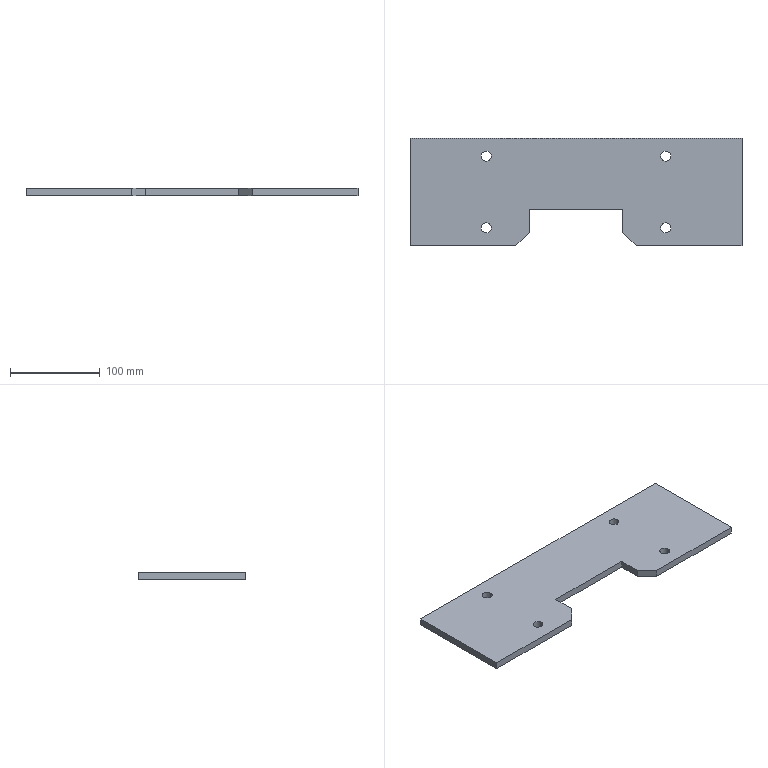Component | SolidWorks | THK-A1021FrontEndConnectingPlate-1 | 1 solid | 20 faces | box 370 x 120 x 8 mm | volume 317079 mm3 | plane 12 | cylinder 8 | commonest cylinder face diameters 11 x8 | material Q235A
build123d program:
from build123d import *

# Parameters (mm, degrees)
BOSS_EXTRUDE1_DEPTH        = 4
F_11_0_11_DIAMETER_HOLE1_D = 11
CHAMFER1_SIZE              = 15


with BuildPart() as part:
    # Sketch1 → Boss-Extrude1 (new, symmetric)
    with BuildSketch(Plane.XY):
        Polygon((-185, 60), (185, 60), (185, -60), (52, -60), (52, -20), (-52, -20), (-52, -60), (-185, -60), align=None)
    extrude(amount=BOSS_EXTRUDE1_DEPTH, both=True)

    # 11.0 _11_ Diameter Hole1 (through all)
    with Locations(Plane.XY.offset(4)):
        with Locations((-100, 40), (100, 40), (-100, -40), (100, -40)):
            Hole(F_11_0_11_DIAMETER_HOLE1_D / 2)

    # Chamfer1
    chamfer1_edges = [part.edges().sort_by_distance(p)[0] for p in [
        (52, -60, 0),
        (-52, -60, 0),
    ]]
    chamfer(chamfer1_edges, length=CHAMFER1_SIZE)


solid = part.part

# Placed as in the assembly
solid = solid.moved(Location((0, -115, -1245), (0, 0, 0)))
STEP:
#1=CARTESIAN_POINT('',(-4.154,-2.953,-49.173));
#2=VERTEX_POINT('',#1);
#3=CARTESIAN_POINT('',(-3.72,-2.953,-49.173));
#4=VERTEX_POINT('',#3);
#5=CARTESIAN_POINT('',(-3.937,-2.953,-49.173));
#6=DIRECTION('',(0.,0.,1.));
#7=DIRECTION('',(1.,0.,0.));
#8=AXIS2_PLACEMENT_3D('',#5,#6,#7);
#9=CIRCLE('',#8,0.2165);
#10=EDGE_CURVE('',#2,#4,#9,.T.);
#11=ORIENTED_EDGE('',*,*,#10,.F.);
#12=CARTESIAN_POINT('',(-4.154,-2.953,-48.858));
#13=VERTEX_POINT('',#12);
#14=CARTESIAN_POINT('',(-4.154,-2.953,-48.858));
#15=DIRECTION('',(0.,0.,1.));
#16=VECTOR('',#15,39.37);
#17=LINE('',#14,#16);
#18=EDGE_CURVE('',#2,#13,#17,.T.);
#19=ORIENTED_EDGE('',*,*,#18,.T.);
#20=CARTESIAN_POINT('',(-3.72,-2.953,-48.858));
#21=VERTEX_POINT('',#20);
#22=CARTESIAN_POINT('',(-3.937,-2.953,-48.858));
#23=DIRECTION('',(0.,0.,1.));
#24=DIRECTION('',(1.,0.,0.));
#25=AXIS2_PLACEMENT_3D('',#22,#23,#24);
#26=CIRCLE('',#25,0.2165);
#27=EDGE_CURVE('',#13,#21,#26,.T.);
#28=ORIENTED_EDGE('',*,*,#27,.T.);
#29=CARTESIAN_POINT('',(-3.72,-2.953,-48.858));
#30=DIRECTION('',(0.,0.,1.));
#31=VECTOR('',#30,39.37);
#32=LINE('',#29,#31);
#33=EDGE_CURVE('',#4,#21,#32,.T.);
#34=ORIENTED_EDGE('',*,*,#33,.F.);
#35=EDGE_LOOP('',(#11,#19,#28,#34));
#36=FACE_OUTER_BOUND('',#35,.T.);
#37=CARTESIAN_POINT('',(-3.937,-2.953,-48.858));
#38=DIRECTION('',(0.,0.,1.));
#39=DIRECTION('',(1.,0.,0.));
#40=AXIS2_PLACEMENT_3D('',#37,#38,#39);
#41=CYLINDRICAL_SURFACE('',#40,0.2165);
#42=ADVANCED_FACE('',(#36),#41,.F.);
#43=CARTESIAN_POINT('',(3.72,-2.953,-49.173));
#44=VERTEX_POINT('',#43);
#45=CARTESIAN_POINT('',(4.154,-2.953,-49.173));
#46=VERTEX_POINT('',#45);
#47=CARTESIAN_POINT('',(3.937,-2.953,-49.173));
#48=DIRECTION('',(0.,0.,1.));
#49=DIRECTION('',(1.,0.,0.));
#50=AXIS2_PLACEMENT_3D('',#47,#48,#49);
#51=CIRCLE('',#50,0.2165);
#52=EDGE_CURVE('',#44,#46,#51,.T.);
#53=ORIENTED_EDGE('',*,*,#52,.F.);
#54=CARTESIAN_POINT('',(3.72,-2.953,-48.858));
#55=VERTEX_POINT('',#54);
#56=CARTESIAN_POINT('',(3.72,-2.953,-48.858));
#57=DIRECTION('',(0.,0.,1.));
#58=VECTOR('',#57,39.37);
#59=LINE('',#56,#58);
#60=EDGE_CURVE('',#44,#55,#59,.T.);
#61=ORIENTED_EDGE('',*,*,#60,.T.);
#62=CARTESIAN_POINT('',(4.154,-2.953,-48.858));
#63=VERTEX_POINT('',#62);
#64=CARTESIAN_POINT('',(3.937,-2.953,-48.858));
#65=DIRECTION('',(0.,0.,1.));
#66=DIRECTION('',(1.,0.,0.));
#67=AXIS2_PLACEMENT_3D('',#64,#65,#66);
#68=CIRCLE('',#67,0.2165);
#69=EDGE_CURVE('',#55,#63,#68,.T.);
#70=ORIENTED_EDGE('',*,*,#69,.T.);
#71=CARTESIAN_POINT('',(4.154,-2.953,-48.858));
#72=DIRECTION('',(0.,0.,1.));
#73=VECTOR('',#72,39.37);
#74=LINE('',#71,#73);
#75=EDGE_CURVE('',#46,#63,#74,.T.);
#76=ORIENTED_EDGE('',*,*,#75,.F.);
#77=EDGE_LOOP('',(#53,#61,#70,#76));
#78=FACE_OUTER_BOUND('',#77,.T.);
#79=CARTESIAN_POINT('',(3.937,-2.953,-48.858));
#80=DIRECTION('',(0.,0.,1.));
#81=DIRECTION('',(1.,0.,0.));
#82=AXIS2_PLACEMENT_3D('',#79,#80,#81);
#83=CYLINDRICAL_SURFACE('',#82,0.2165);
#84=ADVANCED_FACE('',(#78),#83,.F.);
#85=CARTESIAN_POINT('',(-4.154,-6.102,-49.173));
#86=VERTEX_POINT('',#85);
#87=CARTESIAN_POINT('',(-3.72,-6.102,-49.173));
#88=VERTEX_POINT('',#87);
#89=CARTESIAN_POINT('',(-3.937,-6.102,-49.173));
#90=DIRECTION('',(0.,0.,1.));
#91=DIRECTION('',(1.,0.,0.));
#92=AXIS2_PLACEMENT_3D('',#89,#90,#91);
#93=CIRCLE('',#92,0.2165);
#94=EDGE_CURVE('',#86,#88,#93,.T.);
#95=ORIENTED_EDGE('',*,*,#94,.F.);
#96=CARTESIAN_POINT('',(-4.154,-6.102,-48.858));
#97=VERTEX_POINT('',#96);
#98=CARTESIAN_POINT('',(-4.154,-6.102,-48.858));
#99=DIRECTION('',(0.,0.,1.));
#100=VECTOR('',#99,39.37);
#101=LINE('',#98,#100);
#102=EDGE_CURVE('',#86,#97,#101,.T.);
#103=ORIENTED_EDGE('',*,*,#102,.T.);
#104=CARTESIAN_POINT('',(-3.72,-6.102,-48.858));
#105=VERTEX_POINT('',#104);
#106=CARTESIAN_POINT('',(-3.937,-6.102,-48.858));
#107=DIRECTION('',(0.,0.,1.));
#108=DIRECTION('',(1.,0.,0.));
#109=AXIS2_PLACEMENT_3D('',#106,#107,#108);
#110=CIRCLE('',#109,0.2165);
#111=EDGE_CURVE('',#97,#105,#110,.T.);
#112=ORIENTED_EDGE('',*,*,#111,.T.);
#113=CARTESIAN_POINT('',(-3.72,-6.102,-48.858));
#114=DIRECTION('',(0.,0.,1.));
#115=VECTOR('',#114,39.37);
#116=LINE('',#113,#115);
#117=EDGE_CURVE('',#88,#105,#116,.T.);
#118=ORIENTED_EDGE('',*,*,#117,.F.);
#119=EDGE_LOOP('',(#95,#103,#112,#118));
#120=FACE_OUTER_BOUND('',#119,.T.);
#121=CARTESIAN_POINT('',(-3.937,-6.102,-48.858));
#122=DIRECTION('',(0.,0.,1.));
#123=DIRECTION('',(1.,0.,0.));
#124=AXIS2_PLACEMENT_3D('',#121,#122,#123);
#125=CYLINDRICAL_SURFACE('',#124,0.2165);
#126=ADVANCED_FACE('',(#120),#125,.F.);
#127=CARTESIAN_POINT('',(3.72,-6.102,-49.173));
#128=VERTEX_POINT('',#127);
#129=CARTESIAN_POINT('',(4.154,-6.102,-49.173));
#130=VERTEX_POINT('',#129);
#131=CARTESIAN_POINT('',(3.937,-6.102,-49.173));
#132=DIRECTION('',(0.,0.,1.));
#133=DIRECTION('',(1.,0.,0.));
#134=AXIS2_PLACEMENT_3D('',#131,#132,#133);
#135=CIRCLE('',#134,0.2165);
#136=EDGE_CURVE('',#128,#130,#135,.T.);
#137=ORIENTED_EDGE('',*,*,#136,.F.);
#138=CARTESIAN_POINT('',(3.72,-6.102,-48.858));
#139=VERTEX_POINT('',#138);
#140=CARTESIAN_POINT('',(3.72,-6.102,-48.858));
#141=DIRECTION('',(0.,0.,1.));
#142=VECTOR('',#141,39.37);
#143=LINE('',#140,#142);
#144=EDGE_CURVE('',#128,#139,#143,.T.);
#145=ORIENTED_EDGE('',*,*,#144,.T.);
#146=CARTESIAN_POINT('',(4.154,-6.102,-48.858));
#147=VERTEX_POINT('',#146);
#148=CARTESIAN_POINT('',(3.937,-6.102,-48.858));
#149=DIRECTION('',(0.,0.,1.));
#150=DIRECTION('',(1.,0.,0.));
#151=AXIS2_PLACEMENT_3D('',#148,#149,#150);
#152=CIRCLE('',#151,0.2165);
#153=EDGE_CURVE('',#139,#147,#152,.T.);
#154=ORIENTED_EDGE('',*,*,#153,.T.);
#155=CARTESIAN_POINT('',(4.154,-6.102,-48.858));
#156=DIRECTION('',(0.,0.,1.));
#157=VECTOR('',#156,39.37);
#158=LINE('',#155,#157);
#159=EDGE_CURVE('',#130,#147,#158,.T.);
#160=ORIENTED_EDGE('',*,*,#159,.F.);
#161=EDGE_LOOP('',(#137,#145,#154,#160));
#162=FACE_OUTER_BOUND('',#161,.T.);
#163=CARTESIAN_POINT('',(3.937,-6.102,-48.858));
#164=DIRECTION('',(0.,0.,1.));
#165=DIRECTION('',(1.,0.,0.));
#166=AXIS2_PLACEMENT_3D('',#163,#164,#165);
#167=CYLINDRICAL_SURFACE('',#166,0.2165);
#168=ADVANCED_FACE('',(#162),#167,.F.);
#169=CARTESIAN_POINT('',(-7.283,-2.165,-49.173));
#170=VERTEX_POINT('',#169);
#171=CARTESIAN_POINT('',(-7.283,-6.89,-49.173));
#172=VERTEX_POINT('',#171);
#173=CARTESIAN_POINT('',(-7.283,-2.165,-49.173));
#174=DIRECTION('',(0.,-1.,0.));
#175=VECTOR('',#174,39.37);
#176=LINE('',#173,#175);
#177=EDGE_CURVE('',#170,#172,#176,.T.);
#178=ORIENTED_EDGE('',*,*,#177,.T.);
#179=CARTESIAN_POINT('',(-7.283,-6.89,-48.858));
#180=VERTEX_POINT('',#179);
#181=CARTESIAN_POINT('',(-7.283,-6.89,-48.858));
#182=DIRECTION('',(0.,0.,-1.));
#183=VECTOR('',#182,39.37);
#184=LINE('',#181,#183);
#185=EDGE_CURVE('',#180,#172,#184,.T.);
#186=ORIENTED_EDGE('',*,*,#185,.F.);
#187=CARTESIAN_POINT('',(-7.283,-2.165,-48.858));
#188=VERTEX_POINT('',#187);
#189=CARTESIAN_POINT('',(-7.283,-2.165,-48.858));
#190=DIRECTION('',(0.,-1.,0.));
#191=VECTOR('',#190,39.37);
#192=LINE('',#189,#191);
#193=EDGE_CURVE('',#188,#180,#192,.T.);
#194=ORIENTED_EDGE('',*,*,#193,.F.);
#195=CARTESIAN_POINT('',(-7.283,-2.165,-48.858));
#196=DIRECTION('',(0.,0.,-1.));
#197=VECTOR('',#196,39.37);
#198=LINE('',#195,#197);
#199=EDGE_CURVE('',#188,#170,#198,.T.);
#200=ORIENTED_EDGE('',*,*,#199,.T.);
#201=EDGE_LOOP('',(#178,#186,#194,#200));
#202=FACE_OUTER_BOUND('',#201,.T.);
#203=CARTESIAN_POINT('',(-7.283,-2.165,-48.858));
#204=DIRECTION('',(1.,0.,0.));
#205=DIRECTION('',(0.,0.,-1.));
#206=AXIS2_PLACEMENT_3D('',#203,#204,#205);
#207=PLANE('',#206);
#208=ADVANCED_FACE('',(#202),#207,.F.);
#209=CARTESIAN_POINT('',(-2.638,-6.89,-49.173));
#210=VERTEX_POINT('',#209);
#211=CARTESIAN_POINT('',(-7.283,-6.89,-49.173));
#212=DIRECTION('',(1.,-0.,0.));
#213=VECTOR('',#212,39.37);
#214=LINE('',#211,#213);
#215=EDGE_CURVE('',#172,#210,#214,.T.);
#216=ORIENTED_EDGE('',*,*,#215,.T.);
#217=CARTESIAN_POINT('',(-2.638,-6.89,-48.858));
#218=VERTEX_POINT('',#217);
#219=CARTESIAN_POINT('',(-2.638,-6.89,-48.858));
#220=DIRECTION('',(0.,0.,1.));
#221=VECTOR('',#220,39.37);
#222=LINE('',#219,#221);
#223=EDGE_CURVE('',#210,#218,#222,.T.);
#224=ORIENTED_EDGE('',*,*,#223,.T.);
#225=CARTESIAN_POINT('',(-7.283,-6.89,-48.858));
#226=DIRECTION('',(1.,-0.,0.));
#227=VECTOR('',#226,39.37);
#228=LINE('',#225,#227);
#229=EDGE_CURVE('',#180,#218,#228,.T.);
#230=ORIENTED_EDGE('',*,*,#229,.F.);
#231=ORIENTED_EDGE('',*,*,#185,.T.);
#232=EDGE_LOOP('',(#216,#224,#230,#231));
#233=FACE_OUTER_BOUND('',#232,.T.);
#234=CARTESIAN_POINT('',(-7.283,-6.89,-48.858));
#235=DIRECTION('',(0.,1.,0.));
#236=DIRECTION('',(-1.,0.,0.));
#237=AXIS2_PLACEMENT_3D('',#234,#235,#236);
#238=PLANE('',#237);
#239=ADVANCED_FACE('',(#233),#238,.F.);
#240=CARTESIAN_POINT('',(-2.047,-6.299,-48.858));
#241=VERTEX_POINT('',#240);
#242=CARTESIAN_POINT('',(-2.047,-5.315,-48.858));
#243=VERTEX_POINT('',#242);
#244=CARTESIAN_POINT('',(-2.047,-6.89,-48.858));
#245=DIRECTION('',(0.,1.,0.));
#246=VECTOR('',#245,39.37);
#247=LINE('',#244,#246);
#248=EDGE_CURVE('',#241,#243,#247,.T.);
#249=ORIENTED_EDGE('',*,*,#248,.F.);
#250=CARTESIAN_POINT('',(-2.047,-6.299,-49.173));
#251=VERTEX_POINT('',#250);
#252=CARTESIAN_POINT('',(-2.047,-6.299,-48.858));
#253=DIRECTION('',(0.,0.,-1.));
#254=VECTOR('',#253,39.37);
#255=LINE('',#252,#254);
#256=EDGE_CURVE('',#241,#251,#255,.T.);
#257=ORIENTED_EDGE('',*,*,#256,.T.);
#258=CARTESIAN_POINT('',(-2.047,-5.315,-49.173));
#259=VERTEX_POINT('',#258);
#260=CARTESIAN_POINT('',(-2.047,-6.89,-49.173));
#261=DIRECTION('',(0.,1.,0.));
#262=VECTOR('',#261,39.37);
#263=LINE('',#260,#262);
#264=EDGE_CURVE('',#251,#259,#263,.T.);
#265=ORIENTED_EDGE('',*,*,#264,.T.);
#266=CARTESIAN_POINT('',(-2.047,-5.315,-48.858));
#267=DIRECTION('',(0.,0.,-1.));
#268=VECTOR('',#267,39.37);
#269=LINE('',#266,#268);
#270=EDGE_CURVE('',#243,#259,#269,.T.);
#271=ORIENTED_EDGE('',*,*,#270,.F.);
#272=EDGE_LOOP('',(#249,#257,#265,#271));
#273=FACE_OUTER_BOUND('',#272,.T.);
#274=CARTESIAN_POINT('',(-2.047,-6.89,-48.858));
#275=DIRECTION('',(-1.,0.,0.));
#276=DIRECTION('',(0.,0.,1.));
#277=AXIS2_PLACEMENT_3D('',#274,#275,#276);
#278=PLANE('',#277);
#279=ADVANCED_FACE('',(#273),#278,.F.);
#280=CARTESIAN_POINT('',(2.047,-5.315,-49.173));
#281=VERTEX_POINT('',#280);
#282=CARTESIAN_POINT('',(-2.047,-5.315,-49.173));
#283=DIRECTION('',(1.,0.,0.));
#284=VECTOR('',#283,39.37);
#285=LINE('',#282,#284);
#286=EDGE_CURVE('',#259,#281,#285,.T.);
#287=ORIENTED_EDGE('',*,*,#286,.T.);
#288=CARTESIAN_POINT('',(2.047,-5.315,-48.858));
#289=VERTEX_POINT('',#288);
#290=CARTESIAN_POINT('',(2.047,-5.315,-48.858));
#291=DIRECTION('',(0.,0.,-1.));
#292=VECTOR('',#291,39.37);
#293=LINE('',#290,#292);
#294=EDGE_CURVE('',#289,#281,#293,.T.);
#295=ORIENTED_EDGE('',*,*,#294,.F.);
#296=CARTESIAN_POINT('',(-2.047,-5.315,-48.858));
#297=DIRECTION('',(1.,0.,0.));
#298=VECTOR('',#297,39.37);
#299=LINE('',#296,#298);
#300=EDGE_CURVE('',#243,#289,#299,.T.);
#301=ORIENTED_EDGE('',*,*,#300,.F.);
#302=ORIENTED_EDGE('',*,*,#270,.T.);
#303=EDGE_LOOP('',(#287,#295,#301,#302));
#304=FACE_OUTER_BOUND('',#303,.T.);
#305=CARTESIAN_POINT('',(-2.047,-5.315,-48.858));
#306=DIRECTION('',(0.,1.,0.));
#307=DIRECTION('',(0.,0.,1.));
#308=AXIS2_PLACEMENT_3D('',#305,#306,#307);
#309=PLANE('',#308);
#310=ADVANCED_FACE('',(#304),#309,.F.);
#311=CARTESIAN_POINT('',(2.047,-6.299,-49.173));
#312=VERTEX_POINT('',#311);
#313=CARTESIAN_POINT('',(2.047,-6.89,-49.173));
#314=DIRECTION('',(0.,-1.,0.));
#315=VECTOR('',#314,39.37);
#316=LINE('',#313,#315);
#317=EDGE_CURVE('',#281,#312,#316,.T.);
#318=ORIENTED_EDGE('',*,*,#317,.T.);
#319=CARTESIAN_POINT('',(2.047,-6.299,-48.858));
#320=VERTEX_POINT('',#319);
#321=CARTESIAN_POINT('',(2.047,-6.299,-48.858));
#322=DIRECTION('',(0.,0.,1.));
#323=VECTOR('',#322,39.37);
#324=LINE('',#321,#323);
#325=EDGE_CURVE('',#312,#320,#324,.T.);
#326=ORIENTED_EDGE('',*,*,#325,.T.);
#327=CARTESIAN_POINT('',(2.047,-6.89,-48.858));
#328=DIRECTION('',(0.,-1.,0.));
#329=VECTOR('',#328,39.37);
#330=LINE('',#327,#329);
#331=EDGE_CURVE('',#289,#320,#330,.T.);
#332=ORIENTED_EDGE('',*,*,#331,.F.);
#333=ORIENTED_EDGE('',*,*,#294,.T.);
#334=EDGE_LOOP('',(#318,#326,#332,#333));
#335=FACE_OUTER_BOUND('',#334,.T.);
#336=CARTESIAN_POINT('',(2.047,-6.89,-48.858));
#337=DIRECTION('',(1.,0.,0.));
#338=DIRECTION('',(0.,0.,-1.));
#339=AXIS2_PLACEMENT_3D('',#336,#337,#338);
#340=PLANE('',#339);
#341=ADVANCED_FACE('',(#335),#340,.F.);
#342=CARTESIAN_POINT('',(2.638,-6.89,-48.858));
#343=VERTEX_POINT('',#342);
#344=CARTESIAN_POINT('',(7.283,-6.89,-48.858));
#345=VERTEX_POINT('',#344);
#346=CARTESIAN_POINT('',(7.283,-6.89,-48.858));
#347=DIRECTION('',(1.,0.,0.));
#348=VECTOR('',#347,39.37);
#349=LINE('',#346,#348);
#350=EDGE_CURVE('',#343,#345,#349,.T.);
#351=ORIENTED_EDGE('',*,*,#350,.F.);
#352=CARTESIAN_POINT('',(2.638,-6.89,-49.173));
#353=VERTEX_POINT('',#352);
#354=CARTESIAN_POINT('',(2.638,-6.89,-48.858));
#355=DIRECTION('',(0.,0.,-1.));
#356=VECTOR('',#355,39.37);
#357=LINE('',#354,#356);
#358=EDGE_CURVE('',#343,#353,#357,.T.);
#359=ORIENTED_EDGE('',*,*,#358,.T.);
#360=CARTESIAN_POINT('',(7.283,-6.89,-49.173));
#361=VERTEX_POINT('',#360);
#362=CARTESIAN_POINT('',(7.283,-6.89,-49.173));
#363=DIRECTION('',(1.,0.,0.));
#364=VECTOR('',#363,39.37);
#365=LINE('',#362,#364);
#366=EDGE_CURVE('',#353,#361,#365,.T.);
#367=ORIENTED_EDGE('',*,*,#366,.T.);
#368=CARTESIAN_POINT('',(7.283,-6.89,-48.858));
#369=DIRECTION('',(0.,0.,-1.));
#370=VECTOR('',#369,39.37);
#371=LINE('',#368,#370);
#372=EDGE_CURVE('',#345,#361,#371,.T.);
#373=ORIENTED_EDGE('',*,*,#372,.F.);
#374=EDGE_LOOP('',(#351,#359,#367,#373));
#375=FACE_OUTER_BOUND('',#374,.T.);
#376=CARTESIAN_POINT('',(7.283,-6.89,-48.858));
#377=DIRECTION('',(-0.,1.,0.));
#378=DIRECTION('',(-1.,-0.,0.));
#379=AXIS2_PLACEMENT_3D('',#376,#377,#378);
#380=PLANE('',#379);
#381=ADVANCED_FACE('',(#375),#380,.F.);
#382=CARTESIAN_POINT('',(7.283,-2.165,-49.173));
#383=VERTEX_POINT('',#382);
#384=CARTESIAN_POINT('',(7.283,-2.165,-49.173));
#385=DIRECTION('',(0.,1.,0.));
#386=VECTOR('',#385,39.37);
#387=LINE('',#384,#386);
#388=EDGE_CURVE('',#361,#383,#387,.T.);
#389=ORIENTED_EDGE('',*,*,#388,.T.);
#390=CARTESIAN_POINT('',(7.283,-2.165,-48.858));
#391=VERTEX_POINT('',#390);
#392=CARTESIAN_POINT('',(7.283,-2.165,-48.858));
#393=DIRECTION('',(0.,0.,-1.));
#394=VECTOR('',#393,39.37);
#395=LINE('',#392,#394);
#396=EDGE_CURVE('',#391,#383,#395,.T.);
#397=ORIENTED_EDGE('',*,*,#396,.F.);
#398=CARTESIAN_POINT('',(7.283,-2.165,-48.858));
#399=DIRECTION('',(0.,1.,0.));
#400=VECTOR('',#399,39.37);
#401=LINE('',#398,#400);
#402=EDGE_CURVE('',#345,#391,#401,.T.);
#403=ORIENTED_EDGE('',*,*,#402,.F.);
#404=ORIENTED_EDGE('',*,*,#372,.T.);
#405=EDGE_LOOP('',(#389,#397,#403,#404));
#406=FACE_OUTER_BOUND('',#405,.T.);
#407=CARTESIAN_POINT('',(7.283,-2.165,-48.858));
#408=DIRECTION('',(-1.,0.,0.));
#409=DIRECTION('',(0.,0.,1.));
#410=AXIS2_PLACEMENT_3D('',#407,#408,#409);
#411=PLANE('',#410);
#412=ADVANCED_FACE('',(#406),#411,.F.);
#413=CARTESIAN_POINT('',(-7.283,-2.165,-49.173));
#414=DIRECTION('',(-1.,0.,0.));
#415=VECTOR('',#414,39.37);
#416=LINE('',#413,#415);
#417=EDGE_CURVE('',#383,#170,#416,.T.);
#418=ORIENTED_EDGE('',*,*,#417,.T.);
#419=ORIENTED_EDGE('',*,*,#199,.F.);
#420=CARTESIAN_POINT('',(-7.283,-2.165,-48.858));
#421=DIRECTION('',(-1.,0.,0.));
#422=VECTOR('',#421,39.37);
#423=LINE('',#420,#422);
#424=EDGE_CURVE('',#391,#188,#423,.T.);
#425=ORIENTED_EDGE('',*,*,#424,.F.);
#426=ORIENTED_EDGE('',*,*,#396,.T.);
#427=EDGE_LOOP('',(#418,#419,#425,#426));
#428=FACE_OUTER_BOUND('',#427,.T.);
#429=CARTESIAN_POINT('',(-7.283,-2.165,-48.858));
#430=DIRECTION('',(0.,-1.,0.));
#431=DIRECTION('',(0.,0.,-1.));
#432=AXIS2_PLACEMENT_3D('',#429,#430,#431);
#433=PLANE('',#432);
#434=ADVANCED_FACE('',(#428),#433,.F.);
#435=CARTESIAN_POINT('',(-3.937,-2.953,-48.858));
#436=DIRECTION('',(0.,0.,1.));
#437=DIRECTION('',(1.,0.,0.));
#438=AXIS2_PLACEMENT_3D('',#435,#436,#437);
#439=CIRCLE('',#438,0.2165);
#440=EDGE_CURVE('',#21,#13,#439,.T.);
#441=ORIENTED_EDGE('',*,*,#440,.F.);
#442=ORIENTED_EDGE('',*,*,#27,.F.);
#443=EDGE_LOOP('',(#441,#442));
#444=FACE_BOUND('',#443,.T.);
#445=CARTESIAN_POINT('',(3.937,-2.953,-48.858));
#446=DIRECTION('',(0.,0.,1.));
#447=DIRECTION('',(1.,0.,0.));
#448=AXIS2_PLACEMENT_3D('',#445,#446,#447);
#449=CIRCLE('',#448,0.2165);
#450=EDGE_CURVE('',#63,#55,#449,.T.);
#451=ORIENTED_EDGE('',*,*,#450,.F.);
#452=ORIENTED_EDGE('',*,*,#69,.F.);
#453=EDGE_LOOP('',(#451,#452));
#454=FACE_BOUND('',#453,.T.);
#455=CARTESIAN_POINT('',(-3.937,-6.102,-48.858));
#456=DIRECTION('',(0.,0.,1.));
#457=DIRECTION('',(1.,0.,0.));
#458=AXIS2_PLACEMENT_3D('',#455,#456,#457);
#459=CIRCLE('',#458,0.2165);
#460=EDGE_CURVE('',#105,#97,#459,.T.);
#461=ORIENTED_EDGE('',*,*,#460,.F.);
#462=ORIENTED_EDGE('',*,*,#111,.F.);
#463=EDGE_LOOP('',(#461,#462));
#464=FACE_BOUND('',#463,.T.);
#465=CARTESIAN_POINT('',(3.937,-6.102,-48.858));
#466=DIRECTION('',(0.,0.,1.));
#467=DIRECTION('',(1.,0.,0.));
#468=AXIS2_PLACEMENT_3D('',#465,#466,#467);
#469=CIRCLE('',#468,0.2165);
#470=EDGE_CURVE('',#147,#139,#469,.T.);
#471=ORIENTED_EDGE('',*,*,#470,.F.);
#472=ORIENTED_EDGE('',*,*,#153,.F.);
#473=EDGE_LOOP('',(#471,#472));
#474=FACE_BOUND('',#473,.T.);
#475=ORIENTED_EDGE('',*,*,#229,.T.);
#476=CARTESIAN_POINT('',(-0.1378,-4.39,-48.858));
#477=DIRECTION('',(0.7071,0.7071,0.));
#478=VECTOR('',#477,39.37);
#479=LINE('',#476,#478);
#480=EDGE_CURVE('',#218,#241,#479,.T.);
#481=ORIENTED_EDGE('',*,*,#480,.T.);
#482=ORIENTED_EDGE('',*,*,#248,.T.);
#483=ORIENTED_EDGE('',*,*,#300,.T.);
#484=ORIENTED_EDGE('',*,*,#331,.T.);
#485=CARTESIAN_POINT('',(0.1378,-4.39,-48.858));
#486=DIRECTION('',(0.7071,-0.7071,0.));
#487=VECTOR('',#486,39.37);
#488=LINE('',#485,#487);
#489=EDGE_CURVE('',#320,#343,#488,.T.);
#490=ORIENTED_EDGE('',*,*,#489,.T.);
#491=ORIENTED_EDGE('',*,*,#350,.T.);
#492=ORIENTED_EDGE('',*,*,#402,.T.);
#493=ORIENTED_EDGE('',*,*,#424,.T.);
#494=ORIENTED_EDGE('',*,*,#193,.T.);
#495=EDGE_LOOP('',(#475,#481,#482,#483,#484,#490,#491,#492,#493,#494));
#496=FACE_OUTER_BOUND('',#495,.T.);
#497=CARTESIAN_POINT('',(0.,-4.528,-48.858));
#498=DIRECTION('',(0.,0.,1.));
#499=DIRECTION('',(1.,0.,0.));
#500=AXIS2_PLACEMENT_3D('',#497,#498,#499);
#501=PLANE('',#500);
#502=ADVANCED_FACE('',(#444,#454,#464,#474,#496),#501,.T.);
#503=CARTESIAN_POINT('',(-3.937,-2.953,-49.173));
#504=DIRECTION('',(0.,0.,1.));
#505=DIRECTION('',(1.,0.,0.));
#506=AXIS2_PLACEMENT_3D('',#503,#504,#505);
#507=CIRCLE('',#506,0.2165);
#508=EDGE_CURVE('',#4,#2,#507,.T.);
#509=ORIENTED_EDGE('',*,*,#508,.T.);
#510=ORIENTED_EDGE('',*,*,#10,.T.);
#511=EDGE_LOOP('',(#509,#510));
#512=FACE_BOUND('',#511,.T.);
#513=CARTESIAN_POINT('',(3.937,-2.953,-49.173));
#514=DIRECTION('',(0.,0.,1.));
#515=DIRECTION('',(1.,0.,0.));
#516=AXIS2_PLACEMENT_3D('',#513,#514,#515);
#517=CIRCLE('',#516,0.2165);
#518=EDGE_CURVE('',#46,#44,#517,.T.);
#519=ORIENTED_EDGE('',*,*,#518,.T.);
#520=ORIENTED_EDGE('',*,*,#52,.T.);
#521=EDGE_LOOP('',(#519,#520));
#522=FACE_BOUND('',#521,.T.);
#523=CARTESIAN_POINT('',(-3.937,-6.102,-49.173));
#524=DIRECTION('',(0.,0.,1.));
#525=DIRECTION('',(1.,0.,0.));
#526=AXIS2_PLACEMENT_3D('',#523,#524,#525);
#527=CIRCLE('',#526,0.2165);
#528=EDGE_CURVE('',#88,#86,#527,.T.);
#529=ORIENTED_EDGE('',*,*,#528,.T.);
#530=ORIENTED_EDGE('',*,*,#94,.T.);
#531=EDGE_LOOP('',(#529,#530));
#532=FACE_BOUND('',#531,.T.);
#533=CARTESIAN_POINT('',(3.937,-6.102,-49.173));
#534=DIRECTION('',(0.,0.,1.));
#535=DIRECTION('',(1.,0.,0.));
#536=AXIS2_PLACEMENT_3D('',#533,#534,#535);
#537=CIRCLE('',#536,0.2165);
#538=EDGE_CURVE('',#130,#128,#537,.T.);
#539=ORIENTED_EDGE('',*,*,#538,.T.);
#540=ORIENTED_EDGE('',*,*,#136,.T.);
#541=EDGE_LOOP('',(#539,#540));
#542=FACE_BOUND('',#541,.T.);
#543=ORIENTED_EDGE('',*,*,#264,.F.);
#544=CARTESIAN_POINT('',(-2.047,-6.299,-49.173));
#545=DIRECTION('',(-0.7071,-0.7071,0.));
#546=VECTOR('',#545,39.37);
#547=LINE('',#544,#546);
#548=EDGE_CURVE('',#251,#210,#547,.T.);
#549=ORIENTED_EDGE('',*,*,#548,.T.);
#550=ORIENTED_EDGE('',*,*,#215,.F.);
#551=ORIENTED_EDGE('',*,*,#177,.F.);
#552=ORIENTED_EDGE('',*,*,#417,.F.);
#553=ORIENTED_EDGE('',*,*,#388,.F.);
#554=ORIENTED_EDGE('',*,*,#366,.F.);
#555=CARTESIAN_POINT('',(2.638,-6.89,-49.173));
#556=DIRECTION('',(-0.7071,0.7071,0.));
#557=VECTOR('',#556,39.37);
#558=LINE('',#555,#557);
#559=EDGE_CURVE('',#353,#312,#558,.T.);
#560=ORIENTED_EDGE('',*,*,#559,.T.);
#561=ORIENTED_EDGE('',*,*,#317,.F.);
#562=ORIENTED_EDGE('',*,*,#286,.F.);
#563=EDGE_LOOP('',(#543,#549,#550,#551,#552,#553,#554,#560,#561,#562));
#564=FACE_OUTER_BOUND('',#563,.T.);
#565=CARTESIAN_POINT('',(0.,-4.528,-49.173));
#566=DIRECTION('',(0.,0.,1.));
#567=DIRECTION('',(1.,0.,0.));
#568=AXIS2_PLACEMENT_3D('',#565,#566,#567);
#569=PLANE('',#568);
#570=ADVANCED_FACE('',(#512,#522,#532,#542,#564),#569,.F.);
#571=ORIENTED_EDGE('',*,*,#144,.F.);
#572=ORIENTED_EDGE('',*,*,#538,.F.);
#573=ORIENTED_EDGE('',*,*,#159,.T.);
#574=ORIENTED_EDGE('',*,*,#470,.T.);
#575=EDGE_LOOP('',(#571,#572,#573,#574));
#576=FACE_OUTER_BOUND('',#575,.T.);
#577=CARTESIAN_POINT('',(3.937,-6.102,-48.858));
#578=DIRECTION('',(0.,0.,1.));
#579=DIRECTION('',(1.,0.,0.));
#580=AXIS2_PLACEMENT_3D('',#577,#578,#579);
#581=CYLINDRICAL_SURFACE('',#580,0.2165);
#582=ADVANCED_FACE('',(#576),#581,.F.);
#583=ORIENTED_EDGE('',*,*,#102,.F.);
#584=ORIENTED_EDGE('',*,*,#528,.F.);
#585=ORIENTED_EDGE('',*,*,#117,.T.);
#586=ORIENTED_EDGE('',*,*,#460,.T.);
#587=EDGE_LOOP('',(#583,#584,#585,#586));
#588=FACE_OUTER_BOUND('',#587,.T.);
#589=CARTESIAN_POINT('',(-3.937,-6.102,-48.858));
#590=DIRECTION('',(0.,0.,1.));
#591=DIRECTION('',(1.,0.,0.));
#592=AXIS2_PLACEMENT_3D('',#589,#590,#591);
#593=CYLINDRICAL_SURFACE('',#592,0.2165);
#594=ADVANCED_FACE('',(#588),#593,.F.);
#595=ORIENTED_EDGE('',*,*,#60,.F.);
#596=ORIENTED_EDGE('',*,*,#518,.F.);
#597=ORIENTED_EDGE('',*,*,#75,.T.);
#598=ORIENTED_EDGE('',*,*,#450,.T.);
#599=EDGE_LOOP('',(#595,#596,#597,#598));
#600=FACE_OUTER_BOUND('',#599,.T.);
#601=CARTESIAN_POINT('',(3.937,-2.953,-48.858));
#602=DIRECTION('',(0.,0.,1.));
#603=DIRECTION('',(1.,0.,0.));
#604=AXIS2_PLACEMENT_3D('',#601,#602,#603);
#605=CYLINDRICAL_SURFACE('',#604,0.2165);
#606=ADVANCED_FACE('',(#600),#605,.F.);
#607=ORIENTED_EDGE('',*,*,#18,.F.);
#608=ORIENTED_EDGE('',*,*,#508,.F.);
#609=ORIENTED_EDGE('',*,*,#33,.T.);
#610=ORIENTED_EDGE('',*,*,#440,.T.);
#611=EDGE_LOOP('',(#607,#608,#609,#610));
#612=FACE_OUTER_BOUND('',#611,.T.);
#613=CARTESIAN_POINT('',(-3.937,-2.953,-48.858));
#614=DIRECTION('',(0.,0.,1.));
#615=DIRECTION('',(1.,0.,0.));
#616=AXIS2_PLACEMENT_3D('',#613,#614,#615);
#617=CYLINDRICAL_SURFACE('',#616,0.2165);
#618=ADVANCED_FACE('',(#612),#617,.F.);
#619=ORIENTED_EDGE('',*,*,#480,.F.);
#620=ORIENTED_EDGE('',*,*,#223,.F.);
#621=ORIENTED_EDGE('',*,*,#548,.F.);
#622=ORIENTED_EDGE('',*,*,#256,.F.);
#623=EDGE_LOOP('',(#619,#620,#621,#622));
#624=FACE_OUTER_BOUND('',#623,.T.);
#625=CARTESIAN_POINT('',(-2.047,-6.299,-48.858));
#626=DIRECTION('',(-0.7071,0.7071,0.));
#627=DIRECTION('',(0.,0.,-1.));
#628=AXIS2_PLACEMENT_3D('',#625,#626,#627);
#629=PLANE('',#628);
#630=ADVANCED_FACE('',(#624),#629,.F.);
#631=ORIENTED_EDGE('',*,*,#489,.F.);
#632=ORIENTED_EDGE('',*,*,#325,.F.);
#633=ORIENTED_EDGE('',*,*,#559,.F.);
#634=ORIENTED_EDGE('',*,*,#358,.F.);
#635=EDGE_LOOP('',(#631,#632,#633,#634));
#636=FACE_OUTER_BOUND('',#635,.T.);
#637=CARTESIAN_POINT('',(2.638,-6.89,-48.858));
#638=DIRECTION('',(0.7071,0.7071,0.));
#639=DIRECTION('',(0.,0.,-1.));
#640=AXIS2_PLACEMENT_3D('',#637,#638,#639);
#641=PLANE('',#640);
#642=ADVANCED_FACE('',(#636),#641,.F.);
#643=CLOSED_SHELL('',(#42,#84,#126,#168,#208,#239,#279,#310,#341,#381,#412,#434,#502,#570,#582,#594,#606,#618,#630,#642));
#644=MANIFOLD_SOLID_BREP('',#643);
#645=CARTESIAN_POINT('',(0.,0.,0.));
#646=DIRECTION('',(0.,0.,1.));
#647=DIRECTION('',(1.,0.,0.));
#648=AXIS2_PLACEMENT_3D('',#645,#646,#647);
#649=(LENGTH_UNIT()NAMED_UNIT(*)SI_UNIT($,.METRE.));
#650=LENGTH_MEASURE_WITH_UNIT(LENGTH_MEASURE(0.0254),#649);
#651=DIMENSIONAL_EXPONENTS(1.,0.,0.,0.,0.,0.,0.);
#652=(CONVERSION_BASED_UNIT('',#650)LENGTH_UNIT()NAMED_UNIT(#651));
#653=UNCERTAINTY_MEASURE_WITH_UNIT(LENGTH_MEASURE(0.00001),#652,'','');
#654=(NAMED_UNIT(*)PLANE_ANGLE_UNIT()SI_UNIT($,.RADIAN.));
#655=(NAMED_UNIT(*)SI_UNIT($,.STERADIAN.)SOLID_ANGLE_UNIT());
#656=(GEOMETRIC_REPRESENTATION_CONTEXT(3)GLOBAL_UNCERTAINTY_ASSIGNED_CONTEXT((#653))GLOBAL_UNIT_ASSIGNED_CONTEXT((#652,#654,#655))REPRESENTATION_CONTEXT('',''));
#657=ADVANCED_BREP_SHAPE_REPRESENTATION('',(#644,#648),#656);
#658=COLOUR_RGB('',0.7922,0.8196,0.9333);
#659=FILL_AREA_STYLE_COLOUR('',#658);
#660=FILL_AREA_STYLE('',(#659));
#661=SURFACE_STYLE_FILL_AREA(#660);
#662=SURFACE_SIDE_STYLE('',(#661));
#663=SURFACE_STYLE_USAGE(.BOTH.,#662);
#664=PRESENTATION_STYLE_ASSIGNMENT((#663));
#665=STYLED_ITEM('',(#664),#644);
#666=PRESENTATION_LAYER_ASSIGNMENT('','',(#665));
#667=(LENGTH_UNIT()NAMED_UNIT(*)SI_UNIT($,.METRE.));
#668=LENGTH_MEASURE_WITH_UNIT(LENGTH_MEASURE(0.0254),#667);
#669=DIMENSIONAL_EXPONENTS(1.,0.,0.,0.,0.,0.,0.);
#670=(CONVERSION_BASED_UNIT('',#668)LENGTH_UNIT()NAMED_UNIT(#669));
#671=UNCERTAINTY_MEASURE_WITH_UNIT(LENGTH_MEASURE(0.00001),#670,'','');
#672=(NAMED_UNIT(*)PLANE_ANGLE_UNIT()SI_UNIT($,.RADIAN.));
#673=(NAMED_UNIT(*)SI_UNIT($,.STERADIAN.)SOLID_ANGLE_UNIT());
#674=(GEOMETRIC_REPRESENTATION_CONTEXT(3)GLOBAL_UNCERTAINTY_ASSIGNED_CONTEXT((#671))GLOBAL_UNIT_ASSIGNED_CONTEXT((#670,#672,#673))REPRESENTATION_CONTEXT('',''));
#675=MECHANICAL_DESIGN_GEOMETRIC_PRESENTATION_REPRESENTATION('',(#665),#674);